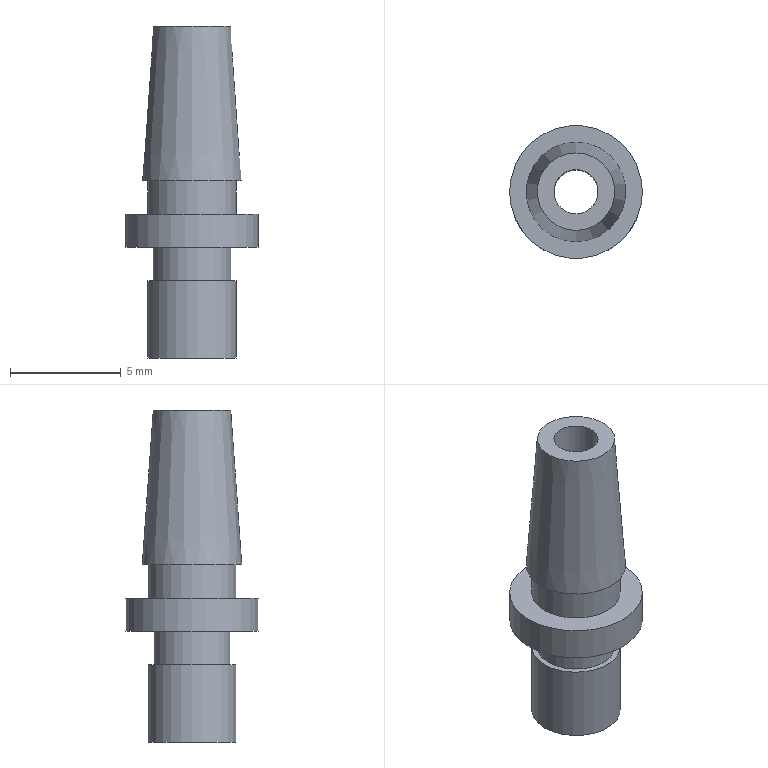Component | NX | PIPE_JOINT | 1 solid | 12 faces | box 6 x 6 x 15 mm | volume 161 mm3 | plane 6 | cylinder 5 | cone 1 | commonest cylinder face diameters 4 x2 3.5 x1 6 x1 2 x1
STEP:
#1=CARTESIAN_POINT('',(0.,0.,0.));
#2=DIRECTION('',(0.,0.,1.));
#3=DIRECTION('',(1.,0.,0.));
#4=AXIS2_PLACEMENT_3D('',#1,#2,#3);
#5=CARTESIAN_POINT('',(13.994,-109.366,22.));
#6=VERTEX_POINT('',#5);
#7=CARTESIAN_POINT('',(13.994,-107.616,22.));
#8=DIRECTION('',(0.,0.,1.));
#9=DIRECTION('',(0.,-1.,0.));
#10=AXIS2_PLACEMENT_3D('',#7,#8,#9);
#11=CIRCLE('',#10,1.75);
#12=CARTESIAN_POINT('',(13.994,-107.616,15.));
#13=DIRECTION('',(0.,0.,-1.));
#14=DIRECTION('',(0.,1.,0.));
#15=AXIS2_PLACEMENT_3D('',#12,#13,#14);
#16=CONICAL_SURFACE('',#15,2.25,0.07131);
#17=CARTESIAN_POINT('',(9.425,-7.));
#18=DIRECTION('',(-1.,0.));
#19=VECTOR('',#18,1.);
#20=LINE('',#17,#19);
#21=(GEOMETRIC_REPRESENTATION_CONTEXT(2)PARAMETRIC_REPRESENTATION_CONTEXT()REPRESENTATION_CONTEXT('',''));
#22=DEFINITIONAL_REPRESENTATION('',(#20),#21);
#23=PCURVE('',#16,#22);
#24=CARTESIAN_POINT('',(13.994,-109.366,22.));
#25=DIRECTION('',(0.,0.,-1.));
#26=DIRECTION('',(0.,1.,0.));
#27=AXIS2_PLACEMENT_3D('',#24,#25,#26);
#28=PLANE('',#27);
#29=CARTESIAN_POINT('',(0.,0.));
#30=CARTESIAN_POINT('',(0.,3.031));
#31=CARTESIAN_POINT('',(2.625,1.516));
#32=CARTESIAN_POINT('',(5.25,0.));
#33=CARTESIAN_POINT('',(2.625,-1.516));
#34=CARTESIAN_POINT('',(0.,-3.031));
#35=CARTESIAN_POINT('',(0.,0.));
#36=(BOUNDED_CURVE()B_SPLINE_CURVE(2,(#29,#30,#31,#32,#33,#34,#35),.UNSPECIFIED.,.T.,.F.)B_SPLINE_CURVE_WITH_KNOTS((1,2,2,2,2,1),(-2.094,0.,2.094,4.189,6.283,8.378),.UNSPECIFIED.)CURVE()GEOMETRIC_REPRESENTATION_ITEM()RATIONAL_B_SPLINE_CURVE((1.,0.5,1.,0.5,1.,0.5,1.))REPRESENTATION_ITEM(''));
#37=(GEOMETRIC_REPRESENTATION_CONTEXT(2)PARAMETRIC_REPRESENTATION_CONTEXT()REPRESENTATION_CONTEXT('',''));
#38=DEFINITIONAL_REPRESENTATION('',(#36),#37);
#39=PCURVE('',#28,#38);
#40=SURFACE_CURVE('',#11,(#23,#39),.PCURVE_S1.);
#41=EDGE_CURVE('',#6,#6,#40,.T.);
#42=ORIENTED_EDGE('',*,*,#41,.F.);
#43=CARTESIAN_POINT('',(13.994,-109.866,15.));
#44=VERTEX_POINT('',#43);
#45=CARTESIAN_POINT('',(13.994,-109.366,22.));
#46=CARTESIAN_POINT('',(13.994,-109.866,15.));
#47=B_SPLINE_CURVE_WITH_KNOTS('',1,(#45,#46),.UNSPECIFIED.,.F.,.F.,(2,2),(-7.018,0.),.PIECEWISE_BEZIER_KNOTS.);
#48=CARTESIAN_POINT('',(9.425,0.));
#49=DIRECTION('',(0.,1.));
#50=VECTOR('',#49,1.);
#51=LINE('',#48,#50);
#52=(GEOMETRIC_REPRESENTATION_CONTEXT(2)PARAMETRIC_REPRESENTATION_CONTEXT()REPRESENTATION_CONTEXT('',''));
#53=DEFINITIONAL_REPRESENTATION('',(#51),#52);
#54=PCURVE('',#16,#53);
#55=CARTESIAN_POINT('',(3.142,0.));
#56=DIRECTION('',(0.,1.));
#57=VECTOR('',#56,1.);
#58=LINE('',#55,#57);
#59=(GEOMETRIC_REPRESENTATION_CONTEXT(2)PARAMETRIC_REPRESENTATION_CONTEXT()REPRESENTATION_CONTEXT('',''));
#60=DEFINITIONAL_REPRESENTATION('',(#58),#59);
#61=PCURVE('',#16,#60);
#62=SEAM_CURVE('',#47,(#54,#61),.PCURVE_S1.);
#63=EDGE_CURVE('',#6,#44,#62,.T.);
#64=ORIENTED_EDGE('',*,*,#63,.T.);
#65=CARTESIAN_POINT('',(13.994,-107.616,15.));
#66=DIRECTION('',(0.,0.,1.));
#67=DIRECTION('',(0.,-1.,0.));
#68=AXIS2_PLACEMENT_3D('',#65,#66,#67);
#69=CIRCLE('',#68,2.25);
#70=CARTESIAN_POINT('',(9.425,0.));
#71=DIRECTION('',(-1.,0.));
#72=VECTOR('',#71,1.);
#73=LINE('',#70,#72);
#74=(GEOMETRIC_REPRESENTATION_CONTEXT(2)PARAMETRIC_REPRESENTATION_CONTEXT()REPRESENTATION_CONTEXT('',''));
#75=DEFINITIONAL_REPRESENTATION('',(#73),#74);
#76=PCURVE('',#16,#75);
#77=CARTESIAN_POINT('',(13.994,-107.616,15.));
#78=DIRECTION('',(0.,0.,1.));
#79=DIRECTION('',(0.,-1.,0.));
#80=AXIS2_PLACEMENT_3D('',#77,#78,#79);
#81=PLANE('',#80);
#82=CARTESIAN_POINT('',(0.,0.));
#83=DIRECTION('',(1.,0.));
#84=AXIS2_PLACEMENT_2D('',#82,#83);
#85=CIRCLE('',#84,2.25);
#86=(GEOMETRIC_REPRESENTATION_CONTEXT(2)PARAMETRIC_REPRESENTATION_CONTEXT()REPRESENTATION_CONTEXT('',''));
#87=DEFINITIONAL_REPRESENTATION('',(#85),#86);
#88=PCURVE('',#81,#87);
#89=SURFACE_CURVE('',#69,(#76,#88),.PCURVE_S1.);
#90=EDGE_CURVE('',#44,#44,#89,.T.);
#91=ORIENTED_EDGE('',*,*,#90,.T.);
#92=ORIENTED_EDGE('',*,*,#63,.F.);
#93=EDGE_LOOP('',(#42,#64,#91,#92));
#94=FACE_BOUND('',#93,.T.);
#95=ADVANCED_FACE('',(#94),#16,.T.);
#96=CARTESIAN_POINT('',(13.994,-106.616,22.));
#97=VERTEX_POINT('',#96);
#98=CARTESIAN_POINT('',(13.994,-107.616,22.));
#99=DIRECTION('',(0.,0.,-1.));
#100=DIRECTION('',(0.,1.,0.));
#101=AXIS2_PLACEMENT_3D('',#98,#99,#100);
#102=CIRCLE('',#101,1.);
#103=CARTESIAN_POINT('',(1.75,0.));
#104=DIRECTION('',(1.,0.));
#105=AXIS2_PLACEMENT_2D('',#103,#104);
#106=CIRCLE('',#105,1.);
#107=(GEOMETRIC_REPRESENTATION_CONTEXT(2)PARAMETRIC_REPRESENTATION_CONTEXT()REPRESENTATION_CONTEXT('',''));
#108=DEFINITIONAL_REPRESENTATION('',(#106),#107);
#109=PCURVE('',#28,#108);
#110=CARTESIAN_POINT('',(13.994,-107.616,107.));
#111=DIRECTION('',(0.,0.,-1.));
#112=DIRECTION('',(0.,1.,0.));
#113=AXIS2_PLACEMENT_3D('',#110,#111,#112);
#114=CYLINDRICAL_SURFACE('',#113,1.);
#115=CARTESIAN_POINT('',(0.,85.));
#116=DIRECTION('',(1.,0.));
#117=VECTOR('',#116,1.);
#118=LINE('',#115,#117);
#119=(GEOMETRIC_REPRESENTATION_CONTEXT(2)PARAMETRIC_REPRESENTATION_CONTEXT()REPRESENTATION_CONTEXT('',''));
#120=DEFINITIONAL_REPRESENTATION('',(#118),#119);
#121=PCURVE('',#114,#120);
#122=SURFACE_CURVE('',#102,(#109,#121),.PCURVE_S1.);
#123=EDGE_CURVE('',#97,#97,#122,.T.);
#124=ORIENTED_EDGE('',*,*,#123,.T.);
#125=EDGE_LOOP('',(#124));
#126=FACE_BOUND('',#125,.T.);
#127=ORIENTED_EDGE('',*,*,#41,.T.);
#128=EDGE_LOOP('',(#127));
#129=FACE_BOUND('',#128,.T.);
#130=ADVANCED_FACE('',(#126,#129),#28,.F.);
#131=CARTESIAN_POINT('',(15.994,-107.616,15.));
#132=VERTEX_POINT('',#131);
#133=CARTESIAN_POINT('',(13.994,-107.616,15.));
#134=DIRECTION('',(0.,0.,1.));
#135=DIRECTION('',(1.,0.,0.));
#136=AXIS2_PLACEMENT_3D('',#133,#134,#135);
#137=CIRCLE('',#136,2.);
#138=CARTESIAN_POINT('',(0.,0.));
#139=DIRECTION('',(0.,1.));
#140=AXIS2_PLACEMENT_2D('',#138,#139);
#141=CIRCLE('',#140,2.);
#142=(GEOMETRIC_REPRESENTATION_CONTEXT(2)PARAMETRIC_REPRESENTATION_CONTEXT()REPRESENTATION_CONTEXT('',''));
#143=DEFINITIONAL_REPRESENTATION('',(#141),#142);
#144=PCURVE('',#81,#143);
#145=CARTESIAN_POINT('',(13.994,-107.616,15.));
#146=DIRECTION('',(0.,0.,-1.));
#147=DIRECTION('',(0.,1.,0.));
#148=AXIS2_PLACEMENT_3D('',#145,#146,#147);
#149=CYLINDRICAL_SURFACE('',#148,2.);
#150=CARTESIAN_POINT('',(7.854,0.));
#151=DIRECTION('',(-1.,0.));
#152=VECTOR('',#151,1.);
#153=LINE('',#150,#152);
#154=(GEOMETRIC_REPRESENTATION_CONTEXT(2)PARAMETRIC_REPRESENTATION_CONTEXT()REPRESENTATION_CONTEXT('',''));
#155=DEFINITIONAL_REPRESENTATION('',(#153),#154);
#156=PCURVE('',#149,#155);
#157=SURFACE_CURVE('',#137,(#144,#156),.PCURVE_S1.);
#158=EDGE_CURVE('',#132,#132,#157,.T.);
#159=ORIENTED_EDGE('',*,*,#158,.T.);
#160=EDGE_LOOP('',(#159));
#161=FACE_BOUND('',#160,.T.);
#162=ORIENTED_EDGE('',*,*,#90,.F.);
#163=EDGE_LOOP('',(#162));
#164=FACE_BOUND('',#163,.T.);
#165=ADVANCED_FACE('',(#161,#164),#81,.F.);
#166=CARTESIAN_POINT('',(15.994,-107.616,7.));
#167=VERTEX_POINT('',#166);
#168=CARTESIAN_POINT('',(13.994,-107.616,7.));
#169=DIRECTION('',(0.,0.,-1.));
#170=DIRECTION('',(1.,0.,0.));
#171=AXIS2_PLACEMENT_3D('',#168,#169,#170);
#172=CIRCLE('',#171,2.);
#173=CARTESIAN_POINT('',(13.994,-107.616,7.));
#174=DIRECTION('',(0.,0.,1.));
#175=DIRECTION('',(0.,-1.,0.));
#176=AXIS2_PLACEMENT_3D('',#173,#174,#175);
#177=CYLINDRICAL_SURFACE('',#176,2.);
#178=CARTESIAN_POINT('',(7.854,0.));
#179=DIRECTION('',(-1.,0.));
#180=VECTOR('',#179,1.);
#181=LINE('',#178,#180);
#182=(GEOMETRIC_REPRESENTATION_CONTEXT(2)PARAMETRIC_REPRESENTATION_CONTEXT()REPRESENTATION_CONTEXT('',''));
#183=DEFINITIONAL_REPRESENTATION('',(#181),#182);
#184=PCURVE('',#177,#183);
#185=CARTESIAN_POINT('',(13.994,-107.616,7.));
#186=DIRECTION('',(0.,0.,-1.));
#187=DIRECTION('',(0.,1.,0.));
#188=AXIS2_PLACEMENT_3D('',#185,#186,#187);
#189=PLANE('',#188);
#190=CARTESIAN_POINT('',(0.,0.));
#191=DIRECTION('',(0.,1.));
#192=AXIS2_PLACEMENT_2D('',#190,#191);
#193=CIRCLE('',#192,2.);
#194=(GEOMETRIC_REPRESENTATION_CONTEXT(2)PARAMETRIC_REPRESENTATION_CONTEXT()REPRESENTATION_CONTEXT('',''));
#195=DEFINITIONAL_REPRESENTATION('',(#193),#194);
#196=PCURVE('',#189,#195);
#197=SURFACE_CURVE('',#172,(#184,#196),.PCURVE_S1.);
#198=EDGE_CURVE('',#167,#167,#197,.T.);
#199=ORIENTED_EDGE('',*,*,#198,.F.);
#200=CARTESIAN_POINT('',(15.994,-107.616,10.5));
#201=VERTEX_POINT('',#200);
#202=CARTESIAN_POINT('',(15.994,-107.616,7.));
#203=CARTESIAN_POINT('',(15.994,-107.616,10.5));
#204=B_SPLINE_CURVE_WITH_KNOTS('',1,(#202,#203),.UNSPECIFIED.,.F.,.F.,(2,2),(0.,3.5),.PIECEWISE_BEZIER_KNOTS.);
#205=CARTESIAN_POINT('',(7.854,0.));
#206=DIRECTION('',(0.,1.));
#207=VECTOR('',#206,1.);
#208=LINE('',#205,#207);
#209=(GEOMETRIC_REPRESENTATION_CONTEXT(2)PARAMETRIC_REPRESENTATION_CONTEXT()REPRESENTATION_CONTEXT('',''));
#210=DEFINITIONAL_REPRESENTATION('',(#208),#209);
#211=PCURVE('',#177,#210);
#212=CARTESIAN_POINT('',(1.571,0.));
#213=DIRECTION('',(0.,1.));
#214=VECTOR('',#213,1.);
#215=LINE('',#212,#214);
#216=(GEOMETRIC_REPRESENTATION_CONTEXT(2)PARAMETRIC_REPRESENTATION_CONTEXT()REPRESENTATION_CONTEXT('',''));
#217=DEFINITIONAL_REPRESENTATION('',(#215),#216);
#218=PCURVE('',#177,#217);
#219=SEAM_CURVE('',#204,(#211,#218),.PCURVE_S1.);
#220=EDGE_CURVE('',#167,#201,#219,.T.);
#221=ORIENTED_EDGE('',*,*,#220,.T.);
#222=CARTESIAN_POINT('',(13.994,-107.616,10.5));
#223=DIRECTION('',(0.,0.,-1.));
#224=DIRECTION('',(1.,0.,0.));
#225=AXIS2_PLACEMENT_3D('',#222,#223,#224);
#226=CIRCLE('',#225,2.);
#227=CARTESIAN_POINT('',(7.854,3.5));
#228=DIRECTION('',(-1.,0.));
#229=VECTOR('',#228,1.);
#230=LINE('',#227,#229);
#231=(GEOMETRIC_REPRESENTATION_CONTEXT(2)PARAMETRIC_REPRESENTATION_CONTEXT()REPRESENTATION_CONTEXT('',''));
#232=DEFINITIONAL_REPRESENTATION('',(#230),#231);
#233=PCURVE('',#177,#232);
#234=CARTESIAN_POINT('',(13.994,-107.616,10.5));
#235=DIRECTION('',(0.,0.,-1.));
#236=DIRECTION('',(0.,1.,0.));
#237=AXIS2_PLACEMENT_3D('',#234,#235,#236);
#238=PLANE('',#237);
#239=CARTESIAN_POINT('',(0.,0.));
#240=DIRECTION('',(0.,1.));
#241=AXIS2_PLACEMENT_2D('',#239,#240);
#242=CIRCLE('',#241,2.);
#243=(GEOMETRIC_REPRESENTATION_CONTEXT(2)PARAMETRIC_REPRESENTATION_CONTEXT()REPRESENTATION_CONTEXT('',''));
#244=DEFINITIONAL_REPRESENTATION('',(#242),#243);
#245=PCURVE('',#238,#244);
#246=SURFACE_CURVE('',#226,(#233,#245),.PCURVE_S1.);
#247=EDGE_CURVE('',#201,#201,#246,.T.);
#248=ORIENTED_EDGE('',*,*,#247,.T.);
#249=ORIENTED_EDGE('',*,*,#220,.F.);
#250=EDGE_LOOP('',(#199,#221,#248,#249));
#251=FACE_BOUND('',#250,.T.);
#252=ADVANCED_FACE('',(#251),#177,.T.);
#253=CARTESIAN_POINT('',(14.994,-107.616,7.));
#254=VERTEX_POINT('',#253);
#255=CARTESIAN_POINT('',(13.994,-106.616,7.));
#256=VERTEX_POINT('',#255);
#257=CARTESIAN_POINT('',(13.994,-107.616,7.));
#258=DIRECTION('',(0.,0.,-1.));
#259=DIRECTION('',(1.,0.,0.));
#260=AXIS2_PLACEMENT_3D('',#257,#258,#259);
#261=CIRCLE('',#260,1.);
#262=CARTESIAN_POINT('',(0.,0.));
#263=DIRECTION('',(0.,1.));
#264=AXIS2_PLACEMENT_2D('',#262,#263);
#265=CIRCLE('',#264,1.);
#266=(GEOMETRIC_REPRESENTATION_CONTEXT(2)PARAMETRIC_REPRESENTATION_CONTEXT()REPRESENTATION_CONTEXT('',''));
#267=DEFINITIONAL_REPRESENTATION('',(#265),#266);
#268=PCURVE('',#189,#267);
#269=CARTESIAN_POINT('',(1.571,100.));
#270=DIRECTION('',(1.,0.));
#271=VECTOR('',#270,1.);
#272=LINE('',#269,#271);
#273=(GEOMETRIC_REPRESENTATION_CONTEXT(2)PARAMETRIC_REPRESENTATION_CONTEXT()REPRESENTATION_CONTEXT('',''));
#274=DEFINITIONAL_REPRESENTATION('',(#272),#273);
#275=PCURVE('',#114,#274);
#276=SURFACE_CURVE('',#261,(#268,#275),.PCURVE_S1.);
#277=EDGE_CURVE('',#254,#256,#276,.T.);
#278=ORIENTED_EDGE('',*,*,#277,.F.);
#279=CARTESIAN_POINT('',(13.994,-107.616,7.));
#280=DIRECTION('',(0.,0.,-1.));
#281=DIRECTION('',(1.,0.,0.));
#282=AXIS2_PLACEMENT_3D('',#279,#280,#281);
#283=CIRCLE('',#282,1.);
#284=CARTESIAN_POINT('',(0.,0.));
#285=DIRECTION('',(0.,1.));
#286=AXIS2_PLACEMENT_2D('',#284,#285);
#287=CIRCLE('',#286,1.);
#288=(GEOMETRIC_REPRESENTATION_CONTEXT(2)PARAMETRIC_REPRESENTATION_CONTEXT()REPRESENTATION_CONTEXT('',''));
#289=DEFINITIONAL_REPRESENTATION('',(#287),#288);
#290=PCURVE('',#189,#289);
#291=CARTESIAN_POINT('',(-4.712,100.));
#292=DIRECTION('',(1.,0.));
#293=VECTOR('',#292,1.);
#294=LINE('',#291,#293);
#295=(GEOMETRIC_REPRESENTATION_CONTEXT(2)PARAMETRIC_REPRESENTATION_CONTEXT()REPRESENTATION_CONTEXT('',''));
#296=DEFINITIONAL_REPRESENTATION('',(#294),#295);
#297=PCURVE('',#114,#296);
#298=SURFACE_CURVE('',#283,(#290,#297),.PCURVE_S1.);
#299=EDGE_CURVE('',#256,#254,#298,.T.);
#300=ORIENTED_EDGE('',*,*,#299,.F.);
#301=EDGE_LOOP('',(#278,#300));
#302=FACE_BOUND('',#301,.T.);
#303=ORIENTED_EDGE('',*,*,#198,.T.);
#304=EDGE_LOOP('',(#303));
#305=FACE_BOUND('',#304,.T.);
#306=ADVANCED_FACE('',(#302,#305),#189,.T.);
#307=CARTESIAN_POINT('',(15.744,-107.616,10.5));
#308=VERTEX_POINT('',#307);
#309=CARTESIAN_POINT('',(13.994,-107.616,10.5));
#310=DIRECTION('',(0.,0.,1.));
#311=DIRECTION('',(1.,0.,0.));
#312=AXIS2_PLACEMENT_3D('',#309,#310,#311);
#313=CIRCLE('',#312,1.75);
#314=CARTESIAN_POINT('',(0.,1.75));
#315=CARTESIAN_POINT('',(3.031,1.75));
#316=CARTESIAN_POINT('',(1.516,-0.875));
#317=CARTESIAN_POINT('',(0.,-3.5));
#318=CARTESIAN_POINT('',(-1.516,-0.875));
#319=CARTESIAN_POINT('',(-3.031,1.75));
#320=CARTESIAN_POINT('',(0.,1.75));
#321=(BOUNDED_CURVE()B_SPLINE_CURVE(2,(#314,#315,#316,#317,#318,#319,#320),.UNSPECIFIED.,.T.,.F.)B_SPLINE_CURVE_WITH_KNOTS((1,2,2,2,2,1),(-2.094,0.,2.094,4.189,6.283,8.378),.UNSPECIFIED.)CURVE()GEOMETRIC_REPRESENTATION_ITEM()RATIONAL_B_SPLINE_CURVE((1.,0.5,1.,0.5,1.,0.5,1.))REPRESENTATION_ITEM(''));
#322=(GEOMETRIC_REPRESENTATION_CONTEXT(2)PARAMETRIC_REPRESENTATION_CONTEXT()REPRESENTATION_CONTEXT('',''));
#323=DEFINITIONAL_REPRESENTATION('',(#321),#322);
#324=PCURVE('',#238,#323);
#325=CARTESIAN_POINT('',(13.994,-107.616,12.));
#326=DIRECTION('',(0.,0.,-1.));
#327=DIRECTION('',(0.,1.,0.));
#328=AXIS2_PLACEMENT_3D('',#325,#326,#327);
#329=CYLINDRICAL_SURFACE('',#328,1.75);
#330=CARTESIAN_POINT('',(7.854,1.5));
#331=DIRECTION('',(-1.,0.));
#332=VECTOR('',#331,1.);
#333=LINE('',#330,#332);
#334=(GEOMETRIC_REPRESENTATION_CONTEXT(2)PARAMETRIC_REPRESENTATION_CONTEXT()REPRESENTATION_CONTEXT('',''));
#335=DEFINITIONAL_REPRESENTATION('',(#333),#334);
#336=PCURVE('',#329,#335);
#337=SURFACE_CURVE('',#313,(#324,#336),.PCURVE_S1.);
#338=EDGE_CURVE('',#308,#308,#337,.T.);
#339=ORIENTED_EDGE('',*,*,#338,.F.);
#340=EDGE_LOOP('',(#339));
#341=FACE_BOUND('',#340,.T.);
#342=ORIENTED_EDGE('',*,*,#247,.F.);
#343=EDGE_LOOP('',(#342));
#344=FACE_BOUND('',#343,.T.);
#345=ADVANCED_FACE('',(#341,#344),#238,.F.);
#346=CARTESIAN_POINT('',(15.744,-107.616,12.));
#347=VERTEX_POINT('',#346);
#348=CARTESIAN_POINT('',(13.994,-107.616,12.));
#349=DIRECTION('',(0.,0.,1.));
#350=DIRECTION('',(1.,0.,0.));
#351=AXIS2_PLACEMENT_3D('',#348,#349,#350);
#352=CIRCLE('',#351,1.75);
#353=CARTESIAN_POINT('',(7.854,0.));
#354=DIRECTION('',(-1.,0.));
#355=VECTOR('',#354,1.);
#356=LINE('',#353,#355);
#357=(GEOMETRIC_REPRESENTATION_CONTEXT(2)PARAMETRIC_REPRESENTATION_CONTEXT()REPRESENTATION_CONTEXT('',''));
#358=DEFINITIONAL_REPRESENTATION('',(#356),#357);
#359=PCURVE('',#329,#358);
#360=CARTESIAN_POINT('',(13.994,-107.616,12.));
#361=DIRECTION('',(0.,0.,1.));
#362=DIRECTION('',(0.,-1.,0.));
#363=AXIS2_PLACEMENT_3D('',#360,#361,#362);
#364=PLANE('',#363);
#365=CARTESIAN_POINT('',(0.,0.));
#366=DIRECTION('',(0.,1.));
#367=AXIS2_PLACEMENT_2D('',#365,#366);
#368=CIRCLE('',#367,1.75);
#369=(GEOMETRIC_REPRESENTATION_CONTEXT(2)PARAMETRIC_REPRESENTATION_CONTEXT()REPRESENTATION_CONTEXT('',''));
#370=DEFINITIONAL_REPRESENTATION('',(#368),#369);
#371=PCURVE('',#364,#370);
#372=SURFACE_CURVE('',#352,(#359,#371),.PCURVE_S1.);
#373=EDGE_CURVE('',#347,#347,#372,.T.);
#374=ORIENTED_EDGE('',*,*,#373,.F.);
#375=CARTESIAN_POINT('',(15.744,-107.616,12.));
#376=CARTESIAN_POINT('',(15.744,-107.616,10.5));
#377=B_SPLINE_CURVE_WITH_KNOTS('',1,(#375,#376),.UNSPECIFIED.,.F.,.F.,(2,2),(0.,1.5),.PIECEWISE_BEZIER_KNOTS.);
#378=CARTESIAN_POINT('',(7.854,0.));
#379=DIRECTION('',(0.,1.));
#380=VECTOR('',#379,1.);
#381=LINE('',#378,#380);
#382=(GEOMETRIC_REPRESENTATION_CONTEXT(2)PARAMETRIC_REPRESENTATION_CONTEXT()REPRESENTATION_CONTEXT('',''));
#383=DEFINITIONAL_REPRESENTATION('',(#381),#382);
#384=PCURVE('',#329,#383);
#385=CARTESIAN_POINT('',(1.571,0.));
#386=DIRECTION('',(0.,1.));
#387=VECTOR('',#386,1.);
#388=LINE('',#385,#387);
#389=(GEOMETRIC_REPRESENTATION_CONTEXT(2)PARAMETRIC_REPRESENTATION_CONTEXT()REPRESENTATION_CONTEXT('',''));
#390=DEFINITIONAL_REPRESENTATION('',(#388),#389);
#391=PCURVE('',#329,#390);
#392=SEAM_CURVE('',#377,(#384,#391),.PCURVE_S1.);
#393=EDGE_CURVE('',#347,#308,#392,.T.);
#394=ORIENTED_EDGE('',*,*,#393,.T.);
#395=ORIENTED_EDGE('',*,*,#338,.T.);
#396=ORIENTED_EDGE('',*,*,#393,.F.);
#397=EDGE_LOOP('',(#374,#394,#395,#396));
#398=FACE_BOUND('',#397,.T.);
#399=ADVANCED_FACE('',(#398),#329,.T.);
#400=CARTESIAN_POINT('',(16.994,-107.616,13.5));
#401=VERTEX_POINT('',#400);
#402=CARTESIAN_POINT('',(13.994,-107.616,13.5));
#403=DIRECTION('',(0.,0.,1.));
#404=DIRECTION('',(1.,0.,0.));
#405=AXIS2_PLACEMENT_3D('',#402,#403,#404);
#406=CIRCLE('',#405,3.);
#407=CARTESIAN_POINT('',(13.994,-107.616,13.5));
#408=DIRECTION('',(0.,0.,-1.));
#409=DIRECTION('',(0.,1.,0.));
#410=AXIS2_PLACEMENT_3D('',#407,#408,#409);
#411=CYLINDRICAL_SURFACE('',#410,3.);
#412=CARTESIAN_POINT('',(7.854,0.));
#413=DIRECTION('',(-1.,0.));
#414=VECTOR('',#413,1.);
#415=LINE('',#412,#414);
#416=(GEOMETRIC_REPRESENTATION_CONTEXT(2)PARAMETRIC_REPRESENTATION_CONTEXT()REPRESENTATION_CONTEXT('',''));
#417=DEFINITIONAL_REPRESENTATION('',(#415),#416);
#418=PCURVE('',#411,#417);
#419=CARTESIAN_POINT('',(13.994,-107.616,13.5));
#420=DIRECTION('',(0.,0.,1.));
#421=DIRECTION('',(0.,-1.,0.));
#422=AXIS2_PLACEMENT_3D('',#419,#420,#421);
#423=PLANE('',#422);
#424=CARTESIAN_POINT('',(0.,0.));
#425=DIRECTION('',(0.,1.));
#426=AXIS2_PLACEMENT_2D('',#424,#425);
#427=CIRCLE('',#426,3.);
#428=(GEOMETRIC_REPRESENTATION_CONTEXT(2)PARAMETRIC_REPRESENTATION_CONTEXT()REPRESENTATION_CONTEXT('',''));
#429=DEFINITIONAL_REPRESENTATION('',(#427),#428);
#430=PCURVE('',#423,#429);
#431=SURFACE_CURVE('',#406,(#418,#430),.PCURVE_S1.);
#432=EDGE_CURVE('',#401,#401,#431,.T.);
#433=ORIENTED_EDGE('',*,*,#432,.F.);
#434=CARTESIAN_POINT('',(16.994,-107.616,12.));
#435=VERTEX_POINT('',#434);
#436=CARTESIAN_POINT('',(16.994,-107.616,13.5));
#437=CARTESIAN_POINT('',(16.994,-107.616,12.));
#438=B_SPLINE_CURVE_WITH_KNOTS('',1,(#436,#437),.UNSPECIFIED.,.F.,.F.,(2,2),(0.,1.5),.PIECEWISE_BEZIER_KNOTS.);
#439=CARTESIAN_POINT('',(7.854,0.));
#440=DIRECTION('',(0.,1.));
#441=VECTOR('',#440,1.);
#442=LINE('',#439,#441);
#443=(GEOMETRIC_REPRESENTATION_CONTEXT(2)PARAMETRIC_REPRESENTATION_CONTEXT()REPRESENTATION_CONTEXT('',''));
#444=DEFINITIONAL_REPRESENTATION('',(#442),#443);
#445=PCURVE('',#411,#444);
#446=CARTESIAN_POINT('',(1.571,0.));
#447=DIRECTION('',(0.,1.));
#448=VECTOR('',#447,1.);
#449=LINE('',#446,#448);
#450=(GEOMETRIC_REPRESENTATION_CONTEXT(2)PARAMETRIC_REPRESENTATION_CONTEXT()REPRESENTATION_CONTEXT('',''));
#451=DEFINITIONAL_REPRESENTATION('',(#449),#450);
#452=PCURVE('',#411,#451);
#453=SEAM_CURVE('',#438,(#445,#452),.PCURVE_S1.);
#454=EDGE_CURVE('',#401,#435,#453,.T.);
#455=ORIENTED_EDGE('',*,*,#454,.T.);
#456=CARTESIAN_POINT('',(13.994,-107.616,12.));
#457=DIRECTION('',(0.,0.,1.));
#458=DIRECTION('',(1.,0.,0.));
#459=AXIS2_PLACEMENT_3D('',#456,#457,#458);
#460=CIRCLE('',#459,3.);
#461=CARTESIAN_POINT('',(7.854,1.5));
#462=DIRECTION('',(-1.,0.));
#463=VECTOR('',#462,1.);
#464=LINE('',#461,#463);
#465=(GEOMETRIC_REPRESENTATION_CONTEXT(2)PARAMETRIC_REPRESENTATION_CONTEXT()REPRESENTATION_CONTEXT('',''));
#466=DEFINITIONAL_REPRESENTATION('',(#464),#465);
#467=PCURVE('',#411,#466);
#468=CARTESIAN_POINT('',(0.,0.));
#469=DIRECTION('',(0.,1.));
#470=AXIS2_PLACEMENT_2D('',#468,#469);
#471=CIRCLE('',#470,3.);
#472=(GEOMETRIC_REPRESENTATION_CONTEXT(2)PARAMETRIC_REPRESENTATION_CONTEXT()REPRESENTATION_CONTEXT('',''));
#473=DEFINITIONAL_REPRESENTATION('',(#471),#472);
#474=PCURVE('',#364,#473);
#475=SURFACE_CURVE('',#460,(#467,#474),.PCURVE_S1.);
#476=EDGE_CURVE('',#435,#435,#475,.T.);
#477=ORIENTED_EDGE('',*,*,#476,.T.);
#478=ORIENTED_EDGE('',*,*,#454,.F.);
#479=EDGE_LOOP('',(#433,#455,#477,#478));
#480=FACE_BOUND('',#479,.T.);
#481=ADVANCED_FACE('',(#480),#411,.T.);
#482=CARTESIAN_POINT('',(15.994,-107.616,13.5));
#483=VERTEX_POINT('',#482);
#484=CARTESIAN_POINT('',(13.994,-107.616,13.5));
#485=DIRECTION('',(0.,0.,1.));
#486=DIRECTION('',(1.,0.,0.));
#487=AXIS2_PLACEMENT_3D('',#484,#485,#486);
#488=CIRCLE('',#487,2.);
#489=CARTESIAN_POINT('',(0.,0.));
#490=DIRECTION('',(0.,1.));
#491=AXIS2_PLACEMENT_2D('',#489,#490);
#492=CIRCLE('',#491,2.);
#493=(GEOMETRIC_REPRESENTATION_CONTEXT(2)PARAMETRIC_REPRESENTATION_CONTEXT()REPRESENTATION_CONTEXT('',''));
#494=DEFINITIONAL_REPRESENTATION('',(#492),#493);
#495=PCURVE('',#423,#494);
#496=CARTESIAN_POINT('',(7.854,1.5));
#497=DIRECTION('',(-1.,0.));
#498=VECTOR('',#497,1.);
#499=LINE('',#496,#498);
#500=(GEOMETRIC_REPRESENTATION_CONTEXT(2)PARAMETRIC_REPRESENTATION_CONTEXT()REPRESENTATION_CONTEXT('',''));
#501=DEFINITIONAL_REPRESENTATION('',(#499),#500);
#502=PCURVE('',#149,#501);
#503=SURFACE_CURVE('',#488,(#495,#502),.PCURVE_S1.);
#504=EDGE_CURVE('',#483,#483,#503,.T.);
#505=ORIENTED_EDGE('',*,*,#504,.F.);
#506=EDGE_LOOP('',(#505));
#507=FACE_BOUND('',#506,.T.);
#508=ORIENTED_EDGE('',*,*,#432,.T.);
#509=EDGE_LOOP('',(#508));
#510=FACE_BOUND('',#509,.T.);
#511=ADVANCED_FACE('',(#507,#510),#423,.T.);
#512=ORIENTED_EDGE('',*,*,#373,.T.);
#513=EDGE_LOOP('',(#512));
#514=FACE_BOUND('',#513,.T.);
#515=ORIENTED_EDGE('',*,*,#476,.F.);
#516=EDGE_LOOP('',(#515));
#517=FACE_BOUND('',#516,.T.);
#518=ADVANCED_FACE('',(#514,#517),#364,.F.);
#519=ORIENTED_EDGE('',*,*,#158,.F.);
#520=CARTESIAN_POINT('',(15.994,-107.616,15.));
#521=CARTESIAN_POINT('',(15.994,-107.616,13.5));
#522=B_SPLINE_CURVE_WITH_KNOTS('',1,(#520,#521),.UNSPECIFIED.,.F.,.F.,(2,2),(0.,1.5),.PIECEWISE_BEZIER_KNOTS.);
#523=CARTESIAN_POINT('',(7.854,0.));
#524=DIRECTION('',(0.,1.));
#525=VECTOR('',#524,1.);
#526=LINE('',#523,#525);
#527=(GEOMETRIC_REPRESENTATION_CONTEXT(2)PARAMETRIC_REPRESENTATION_CONTEXT()REPRESENTATION_CONTEXT('',''));
#528=DEFINITIONAL_REPRESENTATION('',(#526),#527);
#529=PCURVE('',#149,#528);
#530=CARTESIAN_POINT('',(1.571,0.));
#531=DIRECTION('',(0.,1.));
#532=VECTOR('',#531,1.);
#533=LINE('',#530,#532);
#534=(GEOMETRIC_REPRESENTATION_CONTEXT(2)PARAMETRIC_REPRESENTATION_CONTEXT()REPRESENTATION_CONTEXT('',''));
#535=DEFINITIONAL_REPRESENTATION('',(#533),#534);
#536=PCURVE('',#149,#535);
#537=SEAM_CURVE('',#522,(#529,#536),.PCURVE_S1.);
#538=EDGE_CURVE('',#132,#483,#537,.T.);
#539=ORIENTED_EDGE('',*,*,#538,.T.);
#540=ORIENTED_EDGE('',*,*,#504,.T.);
#541=ORIENTED_EDGE('',*,*,#538,.F.);
#542=EDGE_LOOP('',(#519,#539,#540,#541));
#543=FACE_BOUND('',#542,.T.);
#544=ADVANCED_FACE('',(#543),#149,.T.);
#545=ORIENTED_EDGE('',*,*,#299,.F.);
#546=CARTESIAN_POINT('',(13.994,-106.616,22.));
#547=CARTESIAN_POINT('',(13.994,-106.616,7.));
#548=B_SPLINE_CURVE_WITH_KNOTS('',1,(#546,#547),.UNSPECIFIED.,.F.,.F.,(2,2),(85.,100.),.PIECEWISE_BEZIER_KNOTS.);
#549=CARTESIAN_POINT('',(0.,0.));
#550=DIRECTION('',(0.,1.));
#551=VECTOR('',#550,1.);
#552=LINE('',#549,#551);
#553=(GEOMETRIC_REPRESENTATION_CONTEXT(2)PARAMETRIC_REPRESENTATION_CONTEXT()REPRESENTATION_CONTEXT('',''));
#554=DEFINITIONAL_REPRESENTATION('',(#552),#553);
#555=PCURVE('',#114,#554);
#556=CARTESIAN_POINT('',(6.283,0.));
#557=DIRECTION('',(0.,1.));
#558=VECTOR('',#557,1.);
#559=LINE('',#556,#558);
#560=(GEOMETRIC_REPRESENTATION_CONTEXT(2)PARAMETRIC_REPRESENTATION_CONTEXT()REPRESENTATION_CONTEXT('',''));
#561=DEFINITIONAL_REPRESENTATION('',(#559),#560);
#562=PCURVE('',#114,#561);
#563=SEAM_CURVE('',#548,(#555,#562),.PCURVE_S1.);
#564=EDGE_CURVE('',#97,#256,#563,.T.);
#565=ORIENTED_EDGE('',*,*,#564,.F.);
#566=ORIENTED_EDGE('',*,*,#123,.T.);
#567=ORIENTED_EDGE('',*,*,#564,.T.);
#568=ORIENTED_EDGE('',*,*,#277,.F.);
#569=EDGE_LOOP('',(#545,#565,#566,#567,#568));
#570=FACE_BOUND('',#569,.F.);
#571=ADVANCED_FACE('',(#570),#114,.F.);
#572=CLOSED_SHELL('',(#95,#130,#165,#252,#306,#345,#399,#481,#511,#518,#544,#571));
#573=MANIFOLD_SOLID_BREP('',#572);
#574=(LENGTH_UNIT()NAMED_UNIT(*)SI_UNIT(.MILLI.,.METRE.));
#575=UNCERTAINTY_MEASURE_WITH_UNIT(LENGTH_MEASURE(0.00001),#574,'','');
#576=(NAMED_UNIT(*)PLANE_ANGLE_UNIT()SI_UNIT($,.RADIAN.));
#577=(NAMED_UNIT(*)SI_UNIT($,.STERADIAN.)SOLID_ANGLE_UNIT());
#578=(GEOMETRIC_REPRESENTATION_CONTEXT(3)GLOBAL_UNCERTAINTY_ASSIGNED_CONTEXT((#575))GLOBAL_UNIT_ASSIGNED_CONTEXT((#574,#576,#577))REPRESENTATION_CONTEXT('',''));
#579=ADVANCED_BREP_SHAPE_REPRESENTATION('',(#4,#573),#578);